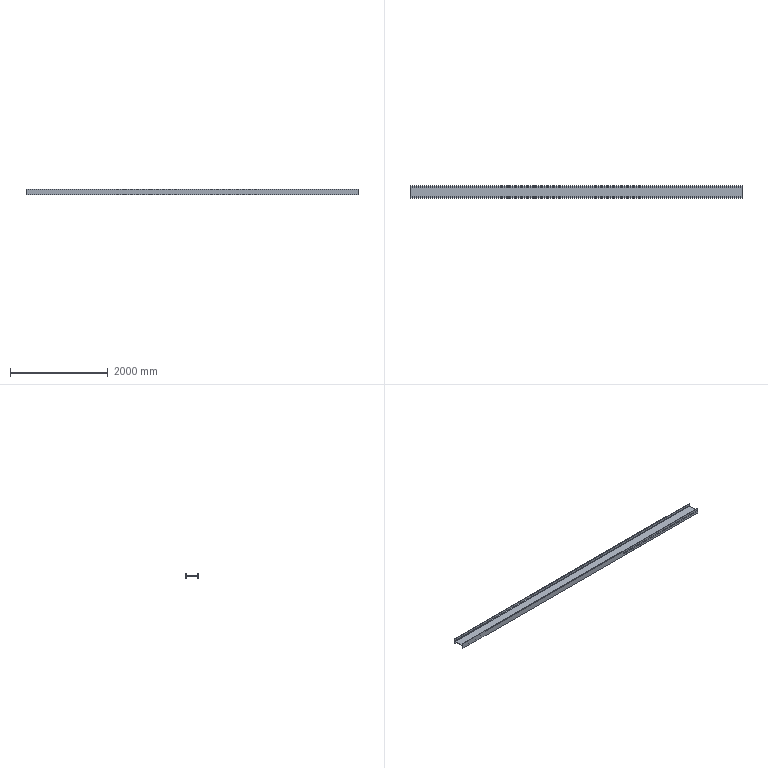Component | NX | P1_2 | 1 solid | 18 faces | volume 33312374 mm3 | plane 14 | cylinder 4 | commonest cylinder face diameters 20 x4